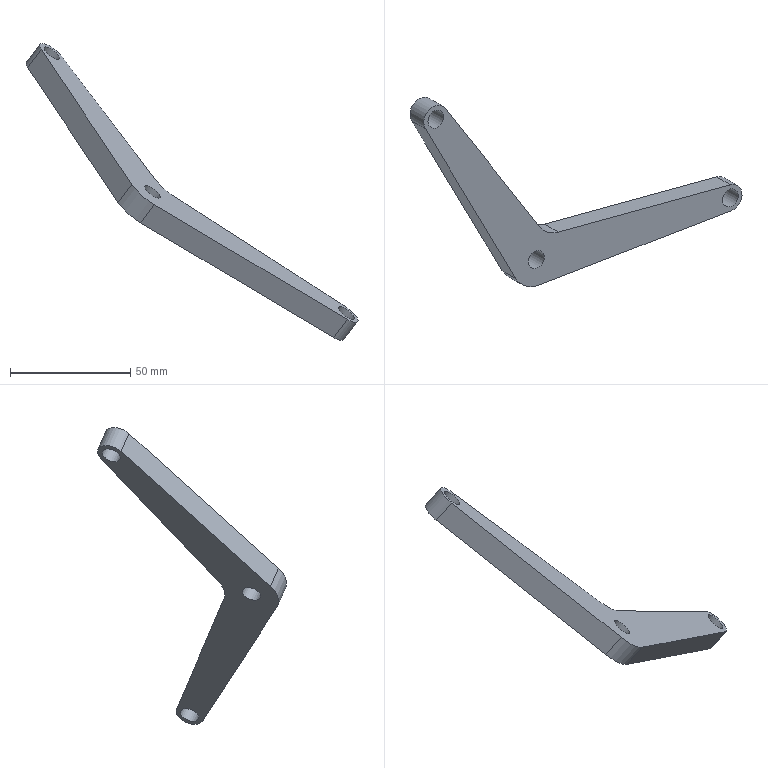Component | NX | QU_BING | 1 solid | 13 faces | box 137.95 x 78.59 x 123.38 mm | volume 32106 mm3 | cylinder 7 | plane 6 | commonest cylinder face diameters 8 x3 24 x2 12.2 x1 11.9 x1
STEP:
#1=CARTESIAN_POINT('',(0.,0.,0.));
#2=DIRECTION('',(0.,0.,1.));
#3=DIRECTION('',(1.,0.,0.));
#4=AXIS2_PLACEMENT_3D('',#1,#2,#3);
#5=CARTESIAN_POINT('',(-160.12,-112.198,24.427));
#6=VERTEX_POINT('',#5);
#7=CARTESIAN_POINT('',(-197.676,-50.115,80.493));
#8=VERTEX_POINT('',#7);
#9=CARTESIAN_POINT('',(-160.12,-112.198,24.427));
#10=DIRECTION('',(-0.4096,0.6771,0.6114));
#11=VECTOR('',#10,1.);
#12=LINE('',#9,#11);
#13=CARTESIAN_POINT('',(-165.855,-108.898,16.93));
#14=DIRECTION('',(0.7094,0.6578,-0.2532));
#15=DIRECTION('',(0.4096,-0.6771,-0.6114));
#16=AXIS2_PLACEMENT_3D('',#13,#14,#15);
#17=PLANE('',#16);
#18=CARTESIAN_POINT('',(0.,-10.));
#19=DIRECTION('',(-1.,-0.));
#20=VECTOR('',#19,1.);
#21=LINE('',#18,#20);
#22=(GEOMETRIC_REPRESENTATION_CONTEXT(2)PARAMETRIC_REPRESENTATION_CONTEXT()REPRESENTATION_CONTEXT('',''));
#23=DEFINITIONAL_REPRESENTATION('',(#21),#22);
#24=PCURVE('',#17,#23);
#25=CARTESIAN_POINT('',(-193.349,-46.103,78.949));
#26=DIRECTION('',(-0.5736,0.3301,-0.7497));
#27=DIRECTION('',(0.7094,0.6578,-0.2532));
#28=AXIS2_PLACEMENT_3D('',#25,#26,#27);
#29=PLANE('',#28);
#30=CARTESIAN_POINT('',(-6.1,91.696));
#31=DIRECTION('',(-0.,-1.));
#32=VECTOR('',#31,1.);
#33=LINE('',#30,#32);
#34=(GEOMETRIC_REPRESENTATION_CONTEXT(2)PARAMETRIC_REPRESENTATION_CONTEXT()REPRESENTATION_CONTEXT('',''));
#35=DEFINITIONAL_REPRESENTATION('',(#33),#34);
#36=PCURVE('',#29,#35);
#37=SURFACE_CURVE('',#12,(#24,#36),.PCURVE_S1.);
#38=EDGE_CURVE('',#6,#8,#37,.T.);
#39=ORIENTED_EDGE('',*,*,#38,.T.);
#40=CARTESIAN_POINT('',(-203.412,-46.814,72.996));
#41=VERTEX_POINT('',#40);
#42=CARTESIAN_POINT('',(-203.412,-46.814,72.996));
#43=DIRECTION('',(0.5736,-0.3301,0.7497));
#44=VECTOR('',#43,1.);
#45=LINE('',#42,#44);
#46=CARTESIAN_POINT('',(-91.696,0.));
#47=DIRECTION('',(0.,-1.));
#48=VECTOR('',#47,1.);
#49=LINE('',#46,#48);
#50=(GEOMETRIC_REPRESENTATION_CONTEXT(2)PARAMETRIC_REPRESENTATION_CONTEXT()REPRESENTATION_CONTEXT('',''));
#51=DEFINITIONAL_REPRESENTATION('',(#49),#50);
#52=PCURVE('',#17,#51);
#53=CARTESIAN_POINT('',(-199.085,-42.802,71.452));
#54=DIRECTION('',(0.5736,-0.3301,0.7497));
#55=DIRECTION('',(-0.7094,-0.6578,0.2532));
#56=AXIS2_PLACEMENT_3D('',#53,#54,#55);
#57=CYLINDRICAL_SURFACE('',#56,6.1);
#58=CARTESIAN_POINT('',(6.283,-0.));
#59=DIRECTION('',(0.,1.));
#60=VECTOR('',#59,1.);
#61=LINE('',#58,#60);
#62=(GEOMETRIC_REPRESENTATION_CONTEXT(2)PARAMETRIC_REPRESENTATION_CONTEXT()REPRESENTATION_CONTEXT('',''));
#63=DEFINITIONAL_REPRESENTATION('',(#61),#62);
#64=PCURVE('',#57,#63);
#65=SURFACE_CURVE('',#45,(#52,#64),.PCURVE_S1.);
#66=EDGE_CURVE('',#41,#8,#65,.T.);
#67=ORIENTED_EDGE('',*,*,#66,.F.);
#68=CARTESIAN_POINT('',(-165.855,-108.898,16.93));
#69=VERTEX_POINT('',#68);
#70=CARTESIAN_POINT('',(-165.855,-108.898,16.93));
#71=DIRECTION('',(-0.4096,0.6771,0.6114));
#72=VECTOR('',#71,1.);
#73=LINE('',#70,#72);
#74=CARTESIAN_POINT('',(0.,0.));
#75=DIRECTION('',(-1.,-0.));
#76=VECTOR('',#75,1.);
#77=LINE('',#74,#76);
#78=(GEOMETRIC_REPRESENTATION_CONTEXT(2)PARAMETRIC_REPRESENTATION_CONTEXT()REPRESENTATION_CONTEXT('',''));
#79=DEFINITIONAL_REPRESENTATION('',(#77),#78);
#80=PCURVE('',#17,#79);
#81=CARTESIAN_POINT('',(-199.085,-42.802,71.452));
#82=DIRECTION('',(-0.5736,0.3301,-0.7497));
#83=DIRECTION('',(0.7094,0.6578,-0.2532));
#84=AXIS2_PLACEMENT_3D('',#81,#82,#83);
#85=PLANE('',#84);
#86=CARTESIAN_POINT('',(-6.1,91.696));
#87=DIRECTION('',(-0.,-1.));
#88=VECTOR('',#87,1.);
#89=LINE('',#86,#88);
#90=(GEOMETRIC_REPRESENTATION_CONTEXT(2)PARAMETRIC_REPRESENTATION_CONTEXT()REPRESENTATION_CONTEXT('',''));
#91=DEFINITIONAL_REPRESENTATION('',(#89),#90);
#92=PCURVE('',#85,#91);
#93=SURFACE_CURVE('',#73,(#80,#92),.PCURVE_S1.);
#94=EDGE_CURVE('',#69,#41,#93,.T.);
#95=ORIENTED_EDGE('',*,*,#94,.F.);
#96=CARTESIAN_POINT('',(-165.855,-108.898,16.93));
#97=DIRECTION('',(0.5736,-0.3301,0.7497));
#98=VECTOR('',#97,1.);
#99=LINE('',#96,#98);
#100=CARTESIAN_POINT('',(0.,0.));
#101=DIRECTION('',(0.,-1.));
#102=VECTOR('',#101,1.);
#103=LINE('',#100,#102);
#104=(GEOMETRIC_REPRESENTATION_CONTEXT(2)PARAMETRIC_REPRESENTATION_CONTEXT()REPRESENTATION_CONTEXT('',''));
#105=DEFINITIONAL_REPRESENTATION('',(#103),#104);
#106=PCURVE('',#17,#105);
#107=CARTESIAN_POINT('',(-157.343,-101.004,13.892));
#108=DIRECTION('',(0.5736,-0.3301,0.7497));
#109=DIRECTION('',(-0.7094,-0.6578,0.2532));
#110=AXIS2_PLACEMENT_3D('',#107,#108,#109);
#111=CYLINDRICAL_SURFACE('',#110,12.);
#112=CARTESIAN_POINT('',(0.,0.));
#113=DIRECTION('',(0.,1.));
#114=VECTOR('',#113,1.);
#115=LINE('',#112,#114);
#116=(GEOMETRIC_REPRESENTATION_CONTEXT(2)PARAMETRIC_REPRESENTATION_CONTEXT()REPRESENTATION_CONTEXT('',''));
#117=DEFINITIONAL_REPRESENTATION('',(#115),#116);
#118=PCURVE('',#111,#117);
#119=SURFACE_CURVE('',#99,(#106,#118),.PCURVE_S1.);
#120=EDGE_CURVE('',#69,#6,#119,.T.);
#121=ORIENTED_EDGE('',*,*,#120,.T.);
#122=EDGE_LOOP('',(#39,#67,#95,#121));
#123=FACE_BOUND('',#122,.T.);
#124=ADVANCED_FACE('',(#123),#17,.F.);
#125=CARTESIAN_POINT('',(-189.306,-41.681,77.803));
#126=VERTEX_POINT('',#125);
#127=CARTESIAN_POINT('',(-193.349,-46.103,78.949));
#128=DIRECTION('',(-0.5736,0.3301,-0.7497));
#129=DIRECTION('',(0.7094,0.6578,-0.2532));
#130=AXIS2_PLACEMENT_3D('',#127,#128,#129);
#131=CIRCLE('',#130,6.1);
#132=CARTESIAN_POINT('',(9.425,10.));
#133=DIRECTION('',(-1.,-0.));
#134=VECTOR('',#133,1.);
#135=LINE('',#132,#134);
#136=(GEOMETRIC_REPRESENTATION_CONTEXT(2)PARAMETRIC_REPRESENTATION_CONTEXT()REPRESENTATION_CONTEXT('',''));
#137=DEFINITIONAL_REPRESENTATION('',(#135),#136);
#138=PCURVE('',#57,#137);
#139=CARTESIAN_POINT('',(0.,0.));
#140=DIRECTION('',(1.,-0.));
#141=AXIS2_PLACEMENT_2D('',#139,#140);
#142=CIRCLE('',#141,6.1);
#143=(GEOMETRIC_REPRESENTATION_CONTEXT(2)PARAMETRIC_REPRESENTATION_CONTEXT()REPRESENTATION_CONTEXT('',''));
#144=DEFINITIONAL_REPRESENTATION('',(#142),#143);
#145=PCURVE('',#29,#144);
#146=SURFACE_CURVE('',#131,(#138,#145),.PCURVE_S1.);
#147=EDGE_CURVE('',#8,#126,#146,.T.);
#148=ORIENTED_EDGE('',*,*,#147,.T.);
#149=CARTESIAN_POINT('',(-195.042,-38.38,70.306));
#150=VERTEX_POINT('',#149);
#151=CARTESIAN_POINT('',(-195.042,-38.38,70.306));
#152=DIRECTION('',(0.5736,-0.3301,0.7497));
#153=VECTOR('',#152,1.);
#154=LINE('',#151,#153);
#155=CARTESIAN_POINT('',(3.246,0.));
#156=DIRECTION('',(0.,1.));
#157=VECTOR('',#156,1.);
#158=LINE('',#155,#157);
#159=(GEOMETRIC_REPRESENTATION_CONTEXT(2)PARAMETRIC_REPRESENTATION_CONTEXT()REPRESENTATION_CONTEXT('',''));
#160=DEFINITIONAL_REPRESENTATION('',(#158),#159);
#161=PCURVE('',#57,#160);
#162=CARTESIAN_POINT('',(-195.042,-38.38,70.306));
#163=DIRECTION('',(-0.6627,-0.7249,0.1879));
#164=DIRECTION('',(-0.4815,0.6046,0.6345));
#165=AXIS2_PLACEMENT_3D('',#162,#163,#164);
#166=PLANE('',#165);
#167=CARTESIAN_POINT('',(0.,0.));
#168=DIRECTION('',(0.,-1.));
#169=VECTOR('',#168,1.);
#170=LINE('',#167,#169);
#171=(GEOMETRIC_REPRESENTATION_CONTEXT(2)PARAMETRIC_REPRESENTATION_CONTEXT()REPRESENTATION_CONTEXT('',''));
#172=DEFINITIONAL_REPRESENTATION('',(#170),#171);
#173=PCURVE('',#166,#172);
#174=SURFACE_CURVE('',#154,(#161,#173),.PCURVE_S1.);
#175=EDGE_CURVE('',#150,#126,#174,.T.);
#176=ORIENTED_EDGE('',*,*,#175,.F.);
#177=CARTESIAN_POINT('',(-199.085,-42.802,71.452));
#178=DIRECTION('',(-0.5736,0.3301,-0.7497));
#179=DIRECTION('',(0.7094,0.6578,-0.2532));
#180=AXIS2_PLACEMENT_3D('',#177,#178,#179);
#181=CIRCLE('',#180,6.1);
#182=CARTESIAN_POINT('',(9.425,0.));
#183=DIRECTION('',(-1.,-0.));
#184=VECTOR('',#183,1.);
#185=LINE('',#182,#184);
#186=(GEOMETRIC_REPRESENTATION_CONTEXT(2)PARAMETRIC_REPRESENTATION_CONTEXT()REPRESENTATION_CONTEXT('',''));
#187=DEFINITIONAL_REPRESENTATION('',(#185),#186);
#188=PCURVE('',#57,#187);
#189=CARTESIAN_POINT('',(0.,0.));
#190=DIRECTION('',(1.,-0.));
#191=AXIS2_PLACEMENT_2D('',#189,#190);
#192=CIRCLE('',#191,6.1);
#193=(GEOMETRIC_REPRESENTATION_CONTEXT(2)PARAMETRIC_REPRESENTATION_CONTEXT()REPRESENTATION_CONTEXT('',''));
#194=DEFINITIONAL_REPRESENTATION('',(#192),#193);
#195=PCURVE('',#85,#194);
#196=SURFACE_CURVE('',#181,(#188,#195),.PCURVE_S1.);
#197=EDGE_CURVE('',#41,#150,#196,.T.);
#198=ORIENTED_EDGE('',*,*,#197,.F.);
#199=ORIENTED_EDGE('',*,*,#66,.T.);
#200=EDGE_LOOP('',(#148,#176,#198,#199));
#201=FACE_BOUND('',#200,.T.);
#202=ADVANCED_FACE('',(#201),#57,.T.);
#203=CARTESIAN_POINT('',(-150.342,-90.607,26.452));
#204=VERTEX_POINT('',#203);
#205=CARTESIAN_POINT('',(-189.306,-41.681,77.803));
#206=DIRECTION('',(0.4815,-0.6046,-0.6345));
#207=VECTOR('',#206,1.);
#208=LINE('',#205,#207);
#209=CARTESIAN_POINT('',(0.,-10.));
#210=DIRECTION('',(-1.,0.));
#211=VECTOR('',#210,1.);
#212=LINE('',#209,#211);
#213=(GEOMETRIC_REPRESENTATION_CONTEXT(2)PARAMETRIC_REPRESENTATION_CONTEXT()REPRESENTATION_CONTEXT('',''));
#214=DEFINITIONAL_REPRESENTATION('',(#212),#213);
#215=PCURVE('',#166,#214);
#216=CARTESIAN_POINT('',(6.067,-0.6376));
#217=DIRECTION('',(0.1045,0.9945));
#218=VECTOR('',#217,1.);
#219=LINE('',#216,#218);
#220=(GEOMETRIC_REPRESENTATION_CONTEXT(2)PARAMETRIC_REPRESENTATION_CONTEXT()REPRESENTATION_CONTEXT('',''));
#221=DEFINITIONAL_REPRESENTATION('',(#219),#220);
#222=PCURVE('',#29,#221);
#223=SURFACE_CURVE('',#208,(#215,#222),.PCURVE_S1.);
#224=EDGE_CURVE('',#126,#204,#223,.T.);
#225=ORIENTED_EDGE('',*,*,#224,.T.);
#226=CARTESIAN_POINT('',(-156.078,-87.306,18.955));
#227=VERTEX_POINT('',#226);
#228=CARTESIAN_POINT('',(-156.078,-87.306,18.955));
#229=DIRECTION('',(0.5736,-0.3301,0.7497));
#230=VECTOR('',#229,1.);
#231=LINE('',#228,#230);
#232=CARTESIAN_POINT('',(-80.925,0.));
#233=DIRECTION('',(0.,-1.));
#234=VECTOR('',#233,1.);
#235=LINE('',#232,#234);
#236=(GEOMETRIC_REPRESENTATION_CONTEXT(2)PARAMETRIC_REPRESENTATION_CONTEXT()REPRESENTATION_CONTEXT('',''));
#237=DEFINITIONAL_REPRESENTATION('',(#235),#236);
#238=PCURVE('',#166,#237);
#239=CARTESIAN_POINT('',(-148.125,-78.607,16.701));
#240=DIRECTION('',(0.5736,-0.3301,0.7497));
#241=DIRECTION('',(-0.7094,-0.6578,0.2532));
#242=AXIS2_PLACEMENT_3D('',#239,#240,#241);
#243=CYLINDRICAL_SURFACE('',#242,12.);
#244=CARTESIAN_POINT('',(0.1047,-0.));
#245=DIRECTION('',(0.,1.));
#246=VECTOR('',#245,1.);
#247=LINE('',#244,#246);
#248=(GEOMETRIC_REPRESENTATION_CONTEXT(2)PARAMETRIC_REPRESENTATION_CONTEXT()REPRESENTATION_CONTEXT('',''));
#249=DEFINITIONAL_REPRESENTATION('',(#247),#248);
#250=PCURVE('',#243,#249);
#251=SURFACE_CURVE('',#231,(#238,#250),.PCURVE_S1.);
#252=EDGE_CURVE('',#227,#204,#251,.T.);
#253=ORIENTED_EDGE('',*,*,#252,.F.);
#254=CARTESIAN_POINT('',(-195.042,-38.38,70.306));
#255=DIRECTION('',(0.4815,-0.6046,-0.6345));
#256=VECTOR('',#255,1.);
#257=LINE('',#254,#256);
#258=CARTESIAN_POINT('',(0.,0.));
#259=DIRECTION('',(-1.,0.));
#260=VECTOR('',#259,1.);
#261=LINE('',#258,#260);
#262=(GEOMETRIC_REPRESENTATION_CONTEXT(2)PARAMETRIC_REPRESENTATION_CONTEXT()REPRESENTATION_CONTEXT('',''));
#263=DEFINITIONAL_REPRESENTATION('',(#261),#262);
#264=PCURVE('',#166,#263);
#265=CARTESIAN_POINT('',(6.067,-0.6376));
#266=DIRECTION('',(0.1045,0.9945));
#267=VECTOR('',#266,1.);
#268=LINE('',#265,#267);
#269=(GEOMETRIC_REPRESENTATION_CONTEXT(2)PARAMETRIC_REPRESENTATION_CONTEXT()REPRESENTATION_CONTEXT('',''));
#270=DEFINITIONAL_REPRESENTATION('',(#268),#269);
#271=PCURVE('',#85,#270);
#272=SURFACE_CURVE('',#257,(#264,#271),.PCURVE_S1.);
#273=EDGE_CURVE('',#150,#227,#272,.T.);
#274=ORIENTED_EDGE('',*,*,#273,.F.);
#275=ORIENTED_EDGE('',*,*,#175,.T.);
#276=EDGE_LOOP('',(#225,#253,#274,#275));
#277=FACE_BOUND('',#276,.T.);
#278=ADVANCED_FACE('',(#277),#166,.F.);
#279=ORIENTED_EDGE('',*,*,#252,.F.);
#280=CARTESIAN_POINT('',(-148.177,-89.604,11.899));
#281=VERTEX_POINT('',#280);
#282=CARTESIAN_POINT('',(-148.125,-78.607,16.701));
#283=DIRECTION('',(0.5736,-0.3301,0.7497));
#284=DIRECTION('',(0.7094,0.6578,-0.2532));
#285=AXIS2_PLACEMENT_3D('',#282,#283,#284);
#286=CIRCLE('',#285,12.);
#287=CARTESIAN_POINT('',(-3.142,-0.));
#288=DIRECTION('',(1.,0.));
#289=VECTOR('',#288,1.);
#290=LINE('',#287,#289);
#291=(GEOMETRIC_REPRESENTATION_CONTEXT(2)PARAMETRIC_REPRESENTATION_CONTEXT()REPRESENTATION_CONTEXT('',''));
#292=DEFINITIONAL_REPRESENTATION('',(#290),#291);
#293=PCURVE('',#243,#292);
#294=CARTESIAN_POINT('',(38.46,78.59));
#295=CARTESIAN_POINT('',(38.46,57.805));
#296=CARTESIAN_POINT('',(20.46,68.198));
#297=CARTESIAN_POINT('',(2.46,78.59));
#298=CARTESIAN_POINT('',(20.46,88.982));
#299=CARTESIAN_POINT('',(38.46,99.375));
#300=CARTESIAN_POINT('',(38.46,78.59));
#301=(BOUNDED_CURVE()B_SPLINE_CURVE(2,(#294,#295,#296,#297,#298,#299,#300),.UNSPECIFIED.,.T.,.F.)B_SPLINE_CURVE_WITH_KNOTS((1,2,2,2,2,1),(-2.094,0.,2.094,4.189,6.283,8.378),.UNSPECIFIED.)CURVE()GEOMETRIC_REPRESENTATION_ITEM()RATIONAL_B_SPLINE_CURVE((1.,0.5,1.,0.5,1.,0.5,1.))REPRESENTATION_ITEM(''));
#302=(GEOMETRIC_REPRESENTATION_CONTEXT(2)PARAMETRIC_REPRESENTATION_CONTEXT()REPRESENTATION_CONTEXT('',''));
#303=DEFINITIONAL_REPRESENTATION('',(#301),#302);
#304=PCURVE('',#85,#303);
#305=SURFACE_CURVE('',#286,(#293,#304),.PCURVE_S1.);
#306=EDGE_CURVE('',#227,#281,#305,.T.);
#307=ORIENTED_EDGE('',*,*,#306,.T.);
#308=CARTESIAN_POINT('',(-142.441,-92.905,19.396));
#309=VERTEX_POINT('',#308);
#310=CARTESIAN_POINT('',(-148.177,-89.604,11.899));
#311=DIRECTION('',(0.5736,-0.3301,0.7497));
#312=VECTOR('',#311,1.);
#313=LINE('',#310,#312);
#314=CARTESIAN_POINT('',(1.042,-0.));
#315=DIRECTION('',(0.,1.));
#316=VECTOR('',#315,1.);
#317=LINE('',#314,#316);
#318=(GEOMETRIC_REPRESENTATION_CONTEXT(2)PARAMETRIC_REPRESENTATION_CONTEXT()REPRESENTATION_CONTEXT('',''));
#319=DEFINITIONAL_REPRESENTATION('',(#317),#318);
#320=PCURVE('',#243,#319);
#321=CARTESIAN_POINT('',(-148.177,-89.604,11.899));
#322=DIRECTION('',(-0.004289,-0.9164,-0.4002));
#323=DIRECTION('',(-0.8191,-0.2263,0.5271));
#324=AXIS2_PLACEMENT_3D('',#321,#322,#323);
#325=PLANE('',#324);
#326=CARTESIAN_POINT('',(0.,0.));
#327=DIRECTION('',(0.,-1.));
#328=VECTOR('',#327,1.);
#329=LINE('',#326,#328);
#330=(GEOMETRIC_REPRESENTATION_CONTEXT(2)PARAMETRIC_REPRESENTATION_CONTEXT()REPRESENTATION_CONTEXT('',''));
#331=DEFINITIONAL_REPRESENTATION('',(#329),#330);
#332=PCURVE('',#325,#331);
#333=SURFACE_CURVE('',#313,(#320,#332),.PCURVE_S1.);
#334=EDGE_CURVE('',#281,#309,#333,.T.);
#335=ORIENTED_EDGE('',*,*,#334,.T.);
#336=CARTESIAN_POINT('',(-142.389,-81.908,24.198));
#337=DIRECTION('',(0.5736,-0.3301,0.7497));
#338=DIRECTION('',(0.7094,0.6578,-0.2532));
#339=AXIS2_PLACEMENT_3D('',#336,#337,#338);
#340=CIRCLE('',#339,12.);
#341=CARTESIAN_POINT('',(-3.142,10.));
#342=DIRECTION('',(1.,0.));
#343=VECTOR('',#342,1.);
#344=LINE('',#341,#343);
#345=(GEOMETRIC_REPRESENTATION_CONTEXT(2)PARAMETRIC_REPRESENTATION_CONTEXT()REPRESENTATION_CONTEXT('',''));
#346=DEFINITIONAL_REPRESENTATION('',(#344),#345);
#347=PCURVE('',#243,#346);
#348=CARTESIAN_POINT('',(38.46,78.59));
#349=CARTESIAN_POINT('',(38.46,57.805));
#350=CARTESIAN_POINT('',(20.46,68.198));
#351=CARTESIAN_POINT('',(2.46,78.59));
#352=CARTESIAN_POINT('',(20.46,88.982));
#353=CARTESIAN_POINT('',(38.46,99.375));
#354=CARTESIAN_POINT('',(38.46,78.59));
#355=(BOUNDED_CURVE()B_SPLINE_CURVE(2,(#348,#349,#350,#351,#352,#353,#354),.UNSPECIFIED.,.T.,.F.)B_SPLINE_CURVE_WITH_KNOTS((1,2,2,2,2,1),(-2.094,0.,2.094,4.189,6.283,8.378),.UNSPECIFIED.)CURVE()GEOMETRIC_REPRESENTATION_ITEM()RATIONAL_B_SPLINE_CURVE((1.,0.5,1.,0.5,1.,0.5,1.))REPRESENTATION_ITEM(''));
#356=(GEOMETRIC_REPRESENTATION_CONTEXT(2)PARAMETRIC_REPRESENTATION_CONTEXT()REPRESENTATION_CONTEXT('',''));
#357=DEFINITIONAL_REPRESENTATION('',(#355),#356);
#358=PCURVE('',#29,#357);
#359=SURFACE_CURVE('',#340,(#347,#358),.PCURVE_S1.);
#360=EDGE_CURVE('',#204,#309,#359,.T.);
#361=ORIENTED_EDGE('',*,*,#360,.F.);
#362=EDGE_LOOP('',(#279,#307,#335,#361));
#363=FACE_BOUND('',#362,.F.);
#364=ADVANCED_FACE('',(#363),#243,.F.);
#365=CARTESIAN_POINT('',(-70.984,-73.162,-26.581));
#366=VERTEX_POINT('',#365);
#367=CARTESIAN_POINT('',(-142.441,-92.905,19.396));
#368=DIRECTION('',(0.8191,0.2263,-0.5271));
#369=VECTOR('',#368,1.);
#370=LINE('',#367,#369);
#371=CARTESIAN_POINT('',(0.,-10.));
#372=DIRECTION('',(-1.,-0.));
#373=VECTOR('',#372,1.);
#374=LINE('',#371,#373);
#375=(GEOMETRIC_REPRESENTATION_CONTEXT(2)PARAMETRIC_REPRESENTATION_CONTEXT()REPRESENTATION_CONTEXT('',''));
#376=DEFINITIONAL_REPRESENTATION('',(#374),#375);
#377=PCURVE('',#325,#376);
#378=CARTESIAN_POINT('',(20.406,88.951));
#379=DIRECTION('',(0.8634,0.5045));
#380=VECTOR('',#379,1.);
#381=LINE('',#378,#380);
#382=(GEOMETRIC_REPRESENTATION_CONTEXT(2)PARAMETRIC_REPRESENTATION_CONTEXT()REPRESENTATION_CONTEXT('',''));
#383=DEFINITIONAL_REPRESENTATION('',(#381),#382);
#384=PCURVE('',#29,#383);
#385=SURFACE_CURVE('',#370,(#377,#384),.PCURVE_S1.);
#386=EDGE_CURVE('',#309,#366,#385,.T.);
#387=ORIENTED_EDGE('',*,*,#386,.T.);
#388=CARTESIAN_POINT('',(-76.72,-69.861,-34.078));
#389=VERTEX_POINT('',#388);
#390=CARTESIAN_POINT('',(-76.72,-69.861,-34.078));
#391=DIRECTION('',(0.5736,-0.3301,0.7497));
#392=VECTOR('',#391,1.);
#393=LINE('',#390,#392);
#394=CARTESIAN_POINT('',(-87.234,0.));
#395=DIRECTION('',(0.,-1.));
#396=VECTOR('',#395,1.);
#397=LINE('',#394,#396);
#398=(GEOMETRIC_REPRESENTATION_CONTEXT(2)PARAMETRIC_REPRESENTATION_CONTEXT()REPRESENTATION_CONTEXT('',''));
#399=DEFINITIONAL_REPRESENTATION('',(#397),#398);
#400=PCURVE('',#325,#399);
#401=CARTESIAN_POINT('',(-76.745,-75.314,-36.459));
#402=DIRECTION('',(0.5736,-0.3301,0.7497));
#403=DIRECTION('',(-0.7094,-0.6578,0.2532));
#404=AXIS2_PLACEMENT_3D('',#401,#402,#403);
#405=CYLINDRICAL_SURFACE('',#404,5.95);
#406=CARTESIAN_POINT('',(4.184,0.));
#407=DIRECTION('',(-0.,1.));
#408=VECTOR('',#407,1.);
#409=LINE('',#406,#408);
#410=(GEOMETRIC_REPRESENTATION_CONTEXT(2)PARAMETRIC_REPRESENTATION_CONTEXT()REPRESENTATION_CONTEXT('',''));
#411=DEFINITIONAL_REPRESENTATION('',(#409),#410);
#412=PCURVE('',#405,#411);
#413=SURFACE_CURVE('',#393,(#400,#412),.PCURVE_S1.);
#414=EDGE_CURVE('',#389,#366,#413,.T.);
#415=ORIENTED_EDGE('',*,*,#414,.F.);
#416=CARTESIAN_POINT('',(-148.177,-89.604,11.899));
#417=DIRECTION('',(0.8191,0.2263,-0.5271));
#418=VECTOR('',#417,1.);
#419=LINE('',#416,#418);
#420=CARTESIAN_POINT('',(0.,0.));
#421=DIRECTION('',(-1.,-0.));
#422=VECTOR('',#421,1.);
#423=LINE('',#420,#422);
#424=(GEOMETRIC_REPRESENTATION_CONTEXT(2)PARAMETRIC_REPRESENTATION_CONTEXT()REPRESENTATION_CONTEXT('',''));
#425=DEFINITIONAL_REPRESENTATION('',(#423),#424);
#426=PCURVE('',#325,#425);
#427=CARTESIAN_POINT('',(20.406,88.951));
#428=DIRECTION('',(0.8634,0.5045));
#429=VECTOR('',#428,1.);
#430=LINE('',#427,#429);
#431=(GEOMETRIC_REPRESENTATION_CONTEXT(2)PARAMETRIC_REPRESENTATION_CONTEXT()REPRESENTATION_CONTEXT('',''));
#432=DEFINITIONAL_REPRESENTATION('',(#430),#431);
#433=PCURVE('',#85,#432);
#434=SURFACE_CURVE('',#419,(#426,#433),.PCURVE_S1.);
#435=EDGE_CURVE('',#281,#389,#434,.T.);
#436=ORIENTED_EDGE('',*,*,#435,.F.);
#437=ORIENTED_EDGE('',*,*,#334,.T.);
#438=EDGE_LOOP('',(#387,#415,#436,#437));
#439=FACE_BOUND('',#438,.T.);
#440=ADVANCED_FACE('',(#439),#325,.F.);
#441=CARTESIAN_POINT('',(-70.551,-83.907,-31.643));
#442=VERTEX_POINT('',#441);
#443=CARTESIAN_POINT('',(-71.01,-78.615,-28.962));
#444=DIRECTION('',(-0.5736,0.3301,-0.7497));
#445=DIRECTION('',(0.7094,0.6578,-0.2532));
#446=AXIS2_PLACEMENT_3D('',#443,#444,#445);
#447=CIRCLE('',#446,5.95);
#448=CARTESIAN_POINT('',(9.425,10.));
#449=DIRECTION('',(-1.,0.));
#450=VECTOR('',#449,1.);
#451=LINE('',#448,#450);
#452=(GEOMETRIC_REPRESENTATION_CONTEXT(2)PARAMETRIC_REPRESENTATION_CONTEXT()REPRESENTATION_CONTEXT('',''));
#453=DEFINITIONAL_REPRESENTATION('',(#451),#452);
#454=PCURVE('',#405,#453);
#455=CARTESIAN_POINT('',(92.721,138.1));
#456=DIRECTION('',(1.,-0.));
#457=AXIS2_PLACEMENT_2D('',#455,#456);
#458=CIRCLE('',#457,5.95);
#459=(GEOMETRIC_REPRESENTATION_CONTEXT(2)PARAMETRIC_REPRESENTATION_CONTEXT()REPRESENTATION_CONTEXT('',''));
#460=DEFINITIONAL_REPRESENTATION('',(#458),#459);
#461=PCURVE('',#29,#460);
#462=SURFACE_CURVE('',#447,(#454,#461),.PCURVE_S1.);
#463=EDGE_CURVE('',#366,#442,#462,.T.);
#464=ORIENTED_EDGE('',*,*,#463,.T.);
#465=CARTESIAN_POINT('',(-76.287,-80.606,-39.14));
#466=VERTEX_POINT('',#465);
#467=CARTESIAN_POINT('',(-76.287,-80.606,-39.14));
#468=DIRECTION('',(0.5736,-0.3301,0.7497));
#469=VECTOR('',#468,1.);
#470=LINE('',#467,#469);
#471=CARTESIAN_POINT('',(1.141,0.));
#472=DIRECTION('',(0.,1.));
#473=VECTOR('',#472,1.);
#474=LINE('',#471,#473);
#475=(GEOMETRIC_REPRESENTATION_CONTEXT(2)PARAMETRIC_REPRESENTATION_CONTEXT()REPRESENTATION_CONTEXT('',''));
#476=DEFINITIONAL_REPRESENTATION('',(#474),#475);
#477=PCURVE('',#405,#476);
#478=CARTESIAN_POINT('',(-76.287,-80.606,-39.14));
#479=DIRECTION('',(-0.07709,0.8894,0.4506));
#480=DIRECTION('',(0.8155,0.3162,-0.4847));
#481=AXIS2_PLACEMENT_3D('',#478,#479,#480);
#482=PLANE('',#481);
#483=CARTESIAN_POINT('',(-0.,0.));
#484=DIRECTION('',(-0.,-1.));
#485=VECTOR('',#484,1.);
#486=LINE('',#483,#485);
#487=(GEOMETRIC_REPRESENTATION_CONTEXT(2)PARAMETRIC_REPRESENTATION_CONTEXT()REPRESENTATION_CONTEXT('',''));
#488=DEFINITIONAL_REPRESENTATION('',(#486),#487);
#489=PCURVE('',#482,#488);
#490=SURFACE_CURVE('',#470,(#477,#489),.PCURVE_S1.);
#491=EDGE_CURVE('',#466,#442,#490,.T.);
#492=ORIENTED_EDGE('',*,*,#491,.F.);
#493=CARTESIAN_POINT('',(-76.745,-75.314,-36.459));
#494=DIRECTION('',(-0.5736,0.3301,-0.7497));
#495=DIRECTION('',(0.7094,0.6578,-0.2532));
#496=AXIS2_PLACEMENT_3D('',#493,#494,#495);
#497=CIRCLE('',#496,5.95);
#498=CARTESIAN_POINT('',(9.425,0.));
#499=DIRECTION('',(-1.,0.));
#500=VECTOR('',#499,1.);
#501=LINE('',#498,#500);
#502=(GEOMETRIC_REPRESENTATION_CONTEXT(2)PARAMETRIC_REPRESENTATION_CONTEXT()REPRESENTATION_CONTEXT('',''));
#503=DEFINITIONAL_REPRESENTATION('',(#501),#502);
#504=PCURVE('',#405,#503);
#505=CARTESIAN_POINT('',(92.721,138.1));
#506=DIRECTION('',(1.,-0.));
#507=AXIS2_PLACEMENT_2D('',#505,#506);
#508=CIRCLE('',#507,5.95);
#509=(GEOMETRIC_REPRESENTATION_CONTEXT(2)PARAMETRIC_REPRESENTATION_CONTEXT()REPRESENTATION_CONTEXT('',''));
#510=DEFINITIONAL_REPRESENTATION('',(#508),#509);
#511=PCURVE('',#85,#510);
#512=SURFACE_CURVE('',#497,(#504,#511),.PCURVE_S1.);
#513=EDGE_CURVE('',#389,#466,#512,.T.);
#514=ORIENTED_EDGE('',*,*,#513,.F.);
#515=ORIENTED_EDGE('',*,*,#414,.T.);
#516=EDGE_LOOP('',(#464,#492,#514,#515));
#517=FACE_BOUND('',#516,.T.);
#518=ADVANCED_FACE('',(#517),#405,.T.);
#519=CARTESIAN_POINT('',(-150.682,-114.978,15.983));
#520=VERTEX_POINT('',#519);
#521=CARTESIAN_POINT('',(-70.551,-83.907,-31.643));
#522=DIRECTION('',(-0.8155,-0.3162,0.4847));
#523=VECTOR('',#522,1.);
#524=LINE('',#521,#523);
#525=CARTESIAN_POINT('',(-0.,-10.));
#526=DIRECTION('',(-1.,0.));
#527=VECTOR('',#526,1.);
#528=LINE('',#525,#527);
#529=(GEOMETRIC_REPRESENTATION_CONTEXT(2)PARAMETRIC_REPRESENTATION_CONTEXT()REPRESENTATION_CONTEXT('',''));
#530=DEFINITIONAL_REPRESENTATION('',(#528),#529);
#531=PCURVE('',#482,#530);
#532=CARTESIAN_POINT('',(90.244,143.51));
#533=DIRECTION('',(-0.9092,-0.4163));
#534=VECTOR('',#533,1.);
#535=LINE('',#532,#534);
#536=(GEOMETRIC_REPRESENTATION_CONTEXT(2)PARAMETRIC_REPRESENTATION_CONTEXT()REPRESENTATION_CONTEXT('',''));
#537=DEFINITIONAL_REPRESENTATION('',(#535),#536);
#538=PCURVE('',#29,#537);
#539=SURFACE_CURVE('',#524,(#531,#538),.PCURVE_S1.);
#540=EDGE_CURVE('',#442,#520,#539,.T.);
#541=ORIENTED_EDGE('',*,*,#540,.T.);
#542=CARTESIAN_POINT('',(-156.417,-111.677,8.486));
#543=VERTEX_POINT('',#542);
#544=CARTESIAN_POINT('',(-156.417,-111.677,8.486));
#545=DIRECTION('',(0.5736,-0.3301,0.7497));
#546=VECTOR('',#545,1.);
#547=LINE('',#544,#546);
#548=CARTESIAN_POINT('',(-98.258,-0.));
#549=DIRECTION('',(-0.,-1.));
#550=VECTOR('',#549,1.);
#551=LINE('',#548,#550);
#552=(GEOMETRIC_REPRESENTATION_CONTEXT(2)PARAMETRIC_REPRESENTATION_CONTEXT()REPRESENTATION_CONTEXT('',''));
#553=DEFINITIONAL_REPRESENTATION('',(#551),#552);
#554=PCURVE('',#482,#553);
#555=CARTESIAN_POINT('',(1.141,0.));
#556=DIRECTION('',(-0.,1.));
#557=VECTOR('',#556,1.);
#558=LINE('',#555,#557);
#559=(GEOMETRIC_REPRESENTATION_CONTEXT(2)PARAMETRIC_REPRESENTATION_CONTEXT()REPRESENTATION_CONTEXT('',''));
#560=DEFINITIONAL_REPRESENTATION('',(#558),#559);
#561=PCURVE('',#111,#560);
#562=SURFACE_CURVE('',#547,(#554,#561),.PCURVE_S1.);
#563=EDGE_CURVE('',#543,#520,#562,.T.);
#564=ORIENTED_EDGE('',*,*,#563,.F.);
#565=CARTESIAN_POINT('',(-76.287,-80.606,-39.14));
#566=DIRECTION('',(-0.8155,-0.3162,0.4847));
#567=VECTOR('',#566,1.);
#568=LINE('',#565,#567);
#569=CARTESIAN_POINT('',(0.,0.));
#570=DIRECTION('',(-1.,0.));
#571=VECTOR('',#570,1.);
#572=LINE('',#569,#571);
#573=(GEOMETRIC_REPRESENTATION_CONTEXT(2)PARAMETRIC_REPRESENTATION_CONTEXT()REPRESENTATION_CONTEXT('',''));
#574=DEFINITIONAL_REPRESENTATION('',(#572),#573);
#575=PCURVE('',#482,#574);
#576=CARTESIAN_POINT('',(90.244,143.51));
#577=DIRECTION('',(-0.9092,-0.4163));
#578=VECTOR('',#577,1.);
#579=LINE('',#576,#578);
#580=(GEOMETRIC_REPRESENTATION_CONTEXT(2)PARAMETRIC_REPRESENTATION_CONTEXT()REPRESENTATION_CONTEXT('',''));
#581=DEFINITIONAL_REPRESENTATION('',(#579),#580);
#582=PCURVE('',#85,#581);
#583=SURFACE_CURVE('',#568,(#575,#582),.PCURVE_S1.);
#584=EDGE_CURVE('',#466,#543,#583,.T.);
#585=ORIENTED_EDGE('',*,*,#584,.F.);
#586=ORIENTED_EDGE('',*,*,#491,.T.);
#587=EDGE_LOOP('',(#541,#564,#585,#586));
#588=FACE_BOUND('',#587,.T.);
#589=ADVANCED_FACE('',(#588),#482,.F.);
#590=CARTESIAN_POINT('',(-154.505,-98.373,12.88));
#591=VERTEX_POINT('',#590);
#592=CARTESIAN_POINT('',(-157.343,-101.004,13.892));
#593=DIRECTION('',(-0.5736,0.3301,-0.7497));
#594=DIRECTION('',(0.7094,0.6578,-0.2532));
#595=AXIS2_PLACEMENT_3D('',#592,#593,#594);
#596=CIRCLE('',#595,4.);
#597=CARTESIAN_POINT('',(-157.343,-101.004,13.892));
#598=DIRECTION('',(0.5736,-0.3301,0.7497));
#599=DIRECTION('',(-0.7094,-0.6578,0.2532));
#600=AXIS2_PLACEMENT_3D('',#597,#598,#599);
#601=CYLINDRICAL_SURFACE('',#600,4.);
#602=CARTESIAN_POINT('',(9.425,0.));
#603=DIRECTION('',(-1.,0.));
#604=VECTOR('',#603,1.);
#605=LINE('',#602,#604);
#606=(GEOMETRIC_REPRESENTATION_CONTEXT(2)PARAMETRIC_REPRESENTATION_CONTEXT()REPRESENTATION_CONTEXT('',''));
#607=DEFINITIONAL_REPRESENTATION('',(#605),#606);
#608=PCURVE('',#601,#607);
#609=CARTESIAN_POINT('',(5.9,91.696));
#610=DIRECTION('',(1.,0.));
#611=AXIS2_PLACEMENT_2D('',#609,#610);
#612=CIRCLE('',#611,4.);
#613=(GEOMETRIC_REPRESENTATION_CONTEXT(2)PARAMETRIC_REPRESENTATION_CONTEXT()REPRESENTATION_CONTEXT('',''));
#614=DEFINITIONAL_REPRESENTATION('',(#612),#613);
#615=PCURVE('',#85,#614);
#616=SURFACE_CURVE('',#596,(#608,#615),.PCURVE_S1.);
#617=EDGE_CURVE('',#591,#591,#616,.T.);
#618=ORIENTED_EDGE('',*,*,#617,.F.);
#619=CARTESIAN_POINT('',(-148.769,-101.674,20.377));
#620=VERTEX_POINT('',#619);
#621=CARTESIAN_POINT('',(-154.505,-98.373,12.88));
#622=CARTESIAN_POINT('',(-148.769,-101.674,20.377));
#623=B_SPLINE_CURVE_WITH_KNOTS('',1,(#621,#622),.UNSPECIFIED.,.F.,.F.,(2,2),(0.,10.),.PIECEWISE_BEZIER_KNOTS.);
#624=CARTESIAN_POINT('',(9.425,0.));
#625=DIRECTION('',(0.,1.));
#626=VECTOR('',#625,1.);
#627=LINE('',#624,#626);
#628=(GEOMETRIC_REPRESENTATION_CONTEXT(2)PARAMETRIC_REPRESENTATION_CONTEXT()REPRESENTATION_CONTEXT('',''));
#629=DEFINITIONAL_REPRESENTATION('',(#627),#628);
#630=PCURVE('',#601,#629);
#631=CARTESIAN_POINT('',(3.142,0.));
#632=DIRECTION('',(0.,1.));
#633=VECTOR('',#632,1.);
#634=LINE('',#631,#633);
#635=(GEOMETRIC_REPRESENTATION_CONTEXT(2)PARAMETRIC_REPRESENTATION_CONTEXT()REPRESENTATION_CONTEXT('',''));
#636=DEFINITIONAL_REPRESENTATION('',(#634),#635);
#637=PCURVE('',#601,#636);
#638=SEAM_CURVE('',#623,(#630,#637),.PCURVE_S1.);
#639=EDGE_CURVE('',#591,#620,#638,.T.);
#640=ORIENTED_EDGE('',*,*,#639,.T.);
#641=CARTESIAN_POINT('',(-151.607,-104.305,21.389));
#642=DIRECTION('',(-0.5736,0.3301,-0.7497));
#643=DIRECTION('',(0.7094,0.6578,-0.2532));
#644=AXIS2_PLACEMENT_3D('',#641,#642,#643);
#645=CIRCLE('',#644,4.);
#646=CARTESIAN_POINT('',(9.425,10.));
#647=DIRECTION('',(-1.,0.));
#648=VECTOR('',#647,1.);
#649=LINE('',#646,#648);
#650=(GEOMETRIC_REPRESENTATION_CONTEXT(2)PARAMETRIC_REPRESENTATION_CONTEXT()REPRESENTATION_CONTEXT('',''));
#651=DEFINITIONAL_REPRESENTATION('',(#649),#650);
#652=PCURVE('',#601,#651);
#653=CARTESIAN_POINT('',(5.9,91.696));
#654=DIRECTION('',(1.,0.));
#655=AXIS2_PLACEMENT_2D('',#653,#654);
#656=CIRCLE('',#655,4.);
#657=(GEOMETRIC_REPRESENTATION_CONTEXT(2)PARAMETRIC_REPRESENTATION_CONTEXT()REPRESENTATION_CONTEXT('',''));
#658=DEFINITIONAL_REPRESENTATION('',(#656),#657);
#659=PCURVE('',#29,#658);
#660=SURFACE_CURVE('',#645,(#652,#659),.PCURVE_S1.);
#661=EDGE_CURVE('',#620,#620,#660,.T.);
#662=ORIENTED_EDGE('',*,*,#661,.T.);
#663=ORIENTED_EDGE('',*,*,#639,.F.);
#664=EDGE_LOOP('',(#618,#640,#662,#663));
#665=FACE_BOUND('',#664,.F.);
#666=ADVANCED_FACE('',(#665),#601,.F.);
#667=CARTESIAN_POINT('',(-196.247,-40.171,70.439));
#668=VERTEX_POINT('',#667);
#669=CARTESIAN_POINT('',(-199.085,-42.802,71.452));
#670=DIRECTION('',(-0.5736,0.3301,-0.7497));
#671=DIRECTION('',(0.7094,0.6578,-0.2532));
#672=AXIS2_PLACEMENT_3D('',#669,#670,#671);
#673=CIRCLE('',#672,4.);
#674=CARTESIAN_POINT('',(-199.085,-42.802,71.452));
#675=DIRECTION('',(0.5736,-0.3301,0.7497));
#676=DIRECTION('',(-0.7094,-0.6578,0.2532));
#677=AXIS2_PLACEMENT_3D('',#674,#675,#676);
#678=CYLINDRICAL_SURFACE('',#677,4.);
#679=CARTESIAN_POINT('',(9.425,0.));
#680=DIRECTION('',(-1.,0.));
#681=VECTOR('',#680,1.);
#682=LINE('',#679,#681);
#683=(GEOMETRIC_REPRESENTATION_CONTEXT(2)PARAMETRIC_REPRESENTATION_CONTEXT()REPRESENTATION_CONTEXT('',''));
#684=DEFINITIONAL_REPRESENTATION('',(#682),#683);
#685=PCURVE('',#678,#684);
#686=CARTESIAN_POINT('',(0.,0.));
#687=DIRECTION('',(1.,0.));
#688=AXIS2_PLACEMENT_2D('',#686,#687);
#689=CIRCLE('',#688,4.);
#690=(GEOMETRIC_REPRESENTATION_CONTEXT(2)PARAMETRIC_REPRESENTATION_CONTEXT()REPRESENTATION_CONTEXT('',''));
#691=DEFINITIONAL_REPRESENTATION('',(#689),#690);
#692=PCURVE('',#85,#691);
#693=SURFACE_CURVE('',#673,(#685,#692),.PCURVE_S1.);
#694=EDGE_CURVE('',#668,#668,#693,.T.);
#695=ORIENTED_EDGE('',*,*,#694,.F.);
#696=CARTESIAN_POINT('',(-190.511,-43.472,77.936));
#697=VERTEX_POINT('',#696);
#698=CARTESIAN_POINT('',(-196.247,-40.171,70.439));
#699=CARTESIAN_POINT('',(-190.511,-43.472,77.936));
#700=B_SPLINE_CURVE_WITH_KNOTS('',1,(#698,#699),.UNSPECIFIED.,.F.,.F.,(2,2),(0.,10.),.PIECEWISE_BEZIER_KNOTS.);
#701=CARTESIAN_POINT('',(9.425,0.));
#702=DIRECTION('',(0.,1.));
#703=VECTOR('',#702,1.);
#704=LINE('',#701,#703);
#705=(GEOMETRIC_REPRESENTATION_CONTEXT(2)PARAMETRIC_REPRESENTATION_CONTEXT()REPRESENTATION_CONTEXT('',''));
#706=DEFINITIONAL_REPRESENTATION('',(#704),#705);
#707=PCURVE('',#678,#706);
#708=CARTESIAN_POINT('',(3.142,0.));
#709=DIRECTION('',(0.,1.));
#710=VECTOR('',#709,1.);
#711=LINE('',#708,#710);
#712=(GEOMETRIC_REPRESENTATION_CONTEXT(2)PARAMETRIC_REPRESENTATION_CONTEXT()REPRESENTATION_CONTEXT('',''));
#713=DEFINITIONAL_REPRESENTATION('',(#711),#712);
#714=PCURVE('',#678,#713);
#715=SEAM_CURVE('',#700,(#707,#714),.PCURVE_S1.);
#716=EDGE_CURVE('',#668,#697,#715,.T.);
#717=ORIENTED_EDGE('',*,*,#716,.T.);
#718=CARTESIAN_POINT('',(-193.349,-46.103,78.949));
#719=DIRECTION('',(-0.5736,0.3301,-0.7497));
#720=DIRECTION('',(0.7094,0.6578,-0.2532));
#721=AXIS2_PLACEMENT_3D('',#718,#719,#720);
#722=CIRCLE('',#721,4.);
#723=CARTESIAN_POINT('',(9.425,10.));
#724=DIRECTION('',(-1.,0.));
#725=VECTOR('',#724,1.);
#726=LINE('',#723,#725);
#727=(GEOMETRIC_REPRESENTATION_CONTEXT(2)PARAMETRIC_REPRESENTATION_CONTEXT()REPRESENTATION_CONTEXT('',''));
#728=DEFINITIONAL_REPRESENTATION('',(#726),#727);
#729=PCURVE('',#678,#728);
#730=CARTESIAN_POINT('',(0.,0.));
#731=DIRECTION('',(1.,0.));
#732=AXIS2_PLACEMENT_2D('',#730,#731);
#733=CIRCLE('',#732,4.);
#734=(GEOMETRIC_REPRESENTATION_CONTEXT(2)PARAMETRIC_REPRESENTATION_CONTEXT()REPRESENTATION_CONTEXT('',''));
#735=DEFINITIONAL_REPRESENTATION('',(#733),#734);
#736=PCURVE('',#29,#735);
#737=SURFACE_CURVE('',#722,(#729,#736),.PCURVE_S1.);
#738=EDGE_CURVE('',#697,#697,#737,.T.);
#739=ORIENTED_EDGE('',*,*,#738,.T.);
#740=ORIENTED_EDGE('',*,*,#716,.F.);
#741=EDGE_LOOP('',(#695,#717,#739,#740));
#742=FACE_BOUND('',#741,.F.);
#743=ADVANCED_FACE('',(#742),#678,.F.);
#744=CARTESIAN_POINT('',(-151.607,-104.305,21.389));
#745=DIRECTION('',(-0.5736,0.3301,-0.7497));
#746=DIRECTION('',(0.7094,0.6578,-0.2532));
#747=AXIS2_PLACEMENT_3D('',#744,#745,#746);
#748=CIRCLE('',#747,12.);
#749=CARTESIAN_POINT('',(3.142,10.));
#750=DIRECTION('',(-1.,-0.));
#751=VECTOR('',#750,1.);
#752=LINE('',#749,#751);
#753=(GEOMETRIC_REPRESENTATION_CONTEXT(2)PARAMETRIC_REPRESENTATION_CONTEXT()REPRESENTATION_CONTEXT('',''));
#754=DEFINITIONAL_REPRESENTATION('',(#752),#753);
#755=PCURVE('',#111,#754);
#756=CARTESIAN_POINT('',(5.9,91.696));
#757=DIRECTION('',(1.,0.));
#758=AXIS2_PLACEMENT_2D('',#756,#757);
#759=CIRCLE('',#758,12.);
#760=(GEOMETRIC_REPRESENTATION_CONTEXT(2)PARAMETRIC_REPRESENTATION_CONTEXT()REPRESENTATION_CONTEXT('',''));
#761=DEFINITIONAL_REPRESENTATION('',(#759),#760);
#762=PCURVE('',#29,#761);
#763=SURFACE_CURVE('',#748,(#755,#762),.PCURVE_S1.);
#764=EDGE_CURVE('',#520,#6,#763,.T.);
#765=ORIENTED_EDGE('',*,*,#764,.T.);
#766=ORIENTED_EDGE('',*,*,#120,.F.);
#767=CARTESIAN_POINT('',(-157.343,-101.004,13.892));
#768=DIRECTION('',(-0.5736,0.3301,-0.7497));
#769=DIRECTION('',(0.7094,0.6578,-0.2532));
#770=AXIS2_PLACEMENT_3D('',#767,#768,#769);
#771=CIRCLE('',#770,12.);
#772=CARTESIAN_POINT('',(3.142,0.));
#773=DIRECTION('',(-1.,-0.));
#774=VECTOR('',#773,1.);
#775=LINE('',#772,#774);
#776=(GEOMETRIC_REPRESENTATION_CONTEXT(2)PARAMETRIC_REPRESENTATION_CONTEXT()REPRESENTATION_CONTEXT('',''));
#777=DEFINITIONAL_REPRESENTATION('',(#775),#776);
#778=PCURVE('',#111,#777);
#779=CARTESIAN_POINT('',(5.9,91.696));
#780=DIRECTION('',(1.,-0.));
#781=AXIS2_PLACEMENT_2D('',#779,#780);
#782=CIRCLE('',#781,12.);
#783=(GEOMETRIC_REPRESENTATION_CONTEXT(2)PARAMETRIC_REPRESENTATION_CONTEXT()REPRESENTATION_CONTEXT('',''));
#784=DEFINITIONAL_REPRESENTATION('',(#782),#783);
#785=PCURVE('',#85,#784);
#786=SURFACE_CURVE('',#771,(#778,#785),.PCURVE_S1.);
#787=EDGE_CURVE('',#543,#69,#786,.T.);
#788=ORIENTED_EDGE('',*,*,#787,.F.);
#789=ORIENTED_EDGE('',*,*,#563,.T.);
#790=EDGE_LOOP('',(#765,#766,#788,#789));
#791=FACE_BOUND('',#790,.T.);
#792=ADVANCED_FACE('',(#791),#111,.T.);
#793=CARTESIAN_POINT('',(-73.908,-72.683,-37.472));
#794=VERTEX_POINT('',#793);
#795=CARTESIAN_POINT('',(-76.745,-75.314,-36.459));
#796=DIRECTION('',(-0.5736,0.3301,-0.7497));
#797=DIRECTION('',(0.7094,0.6578,-0.2532));
#798=AXIS2_PLACEMENT_3D('',#795,#796,#797);
#799=CIRCLE('',#798,4.);
#800=CARTESIAN_POINT('',(-76.745,-75.314,-36.459));
#801=DIRECTION('',(0.5736,-0.3301,0.7497));
#802=DIRECTION('',(-0.7094,-0.6578,0.2532));
#803=AXIS2_PLACEMENT_3D('',#800,#801,#802);
#804=CYLINDRICAL_SURFACE('',#803,4.);
#805=CARTESIAN_POINT('',(9.425,0.));
#806=DIRECTION('',(-1.,0.));
#807=VECTOR('',#806,1.);
#808=LINE('',#805,#807);
#809=(GEOMETRIC_REPRESENTATION_CONTEXT(2)PARAMETRIC_REPRESENTATION_CONTEXT()REPRESENTATION_CONTEXT('',''));
#810=DEFINITIONAL_REPRESENTATION('',(#808),#809);
#811=PCURVE('',#804,#810);
#812=CARTESIAN_POINT('',(92.721,138.1));
#813=DIRECTION('',(1.,0.));
#814=AXIS2_PLACEMENT_2D('',#812,#813);
#815=CIRCLE('',#814,4.);
#816=(GEOMETRIC_REPRESENTATION_CONTEXT(2)PARAMETRIC_REPRESENTATION_CONTEXT()REPRESENTATION_CONTEXT('',''));
#817=DEFINITIONAL_REPRESENTATION('',(#815),#816);
#818=PCURVE('',#85,#817);
#819=SURFACE_CURVE('',#799,(#811,#818),.PCURVE_S1.);
#820=EDGE_CURVE('',#794,#794,#819,.T.);
#821=ORIENTED_EDGE('',*,*,#820,.F.);
#822=CARTESIAN_POINT('',(-68.172,-75.984,-29.975));
#823=VERTEX_POINT('',#822);
#824=CARTESIAN_POINT('',(-73.908,-72.683,-37.472));
#825=CARTESIAN_POINT('',(-68.172,-75.984,-29.975));
#826=B_SPLINE_CURVE_WITH_KNOTS('',1,(#824,#825),.UNSPECIFIED.,.F.,.F.,(2,2),(0.,10.),.PIECEWISE_BEZIER_KNOTS.);
#827=CARTESIAN_POINT('',(9.425,0.));
#828=DIRECTION('',(0.,1.));
#829=VECTOR('',#828,1.);
#830=LINE('',#827,#829);
#831=(GEOMETRIC_REPRESENTATION_CONTEXT(2)PARAMETRIC_REPRESENTATION_CONTEXT()REPRESENTATION_CONTEXT('',''));
#832=DEFINITIONAL_REPRESENTATION('',(#830),#831);
#833=PCURVE('',#804,#832);
#834=CARTESIAN_POINT('',(3.142,0.));
#835=DIRECTION('',(0.,1.));
#836=VECTOR('',#835,1.);
#837=LINE('',#834,#836);
#838=(GEOMETRIC_REPRESENTATION_CONTEXT(2)PARAMETRIC_REPRESENTATION_CONTEXT()REPRESENTATION_CONTEXT('',''));
#839=DEFINITIONAL_REPRESENTATION('',(#837),#838);
#840=PCURVE('',#804,#839);
#841=SEAM_CURVE('',#826,(#833,#840),.PCURVE_S1.);
#842=EDGE_CURVE('',#794,#823,#841,.T.);
#843=ORIENTED_EDGE('',*,*,#842,.T.);
#844=CARTESIAN_POINT('',(-71.01,-78.615,-28.962));
#845=DIRECTION('',(-0.5736,0.3301,-0.7497));
#846=DIRECTION('',(0.7094,0.6578,-0.2532));
#847=AXIS2_PLACEMENT_3D('',#844,#845,#846);
#848=CIRCLE('',#847,4.);
#849=CARTESIAN_POINT('',(9.425,10.));
#850=DIRECTION('',(-1.,0.));
#851=VECTOR('',#850,1.);
#852=LINE('',#849,#851);
#853=(GEOMETRIC_REPRESENTATION_CONTEXT(2)PARAMETRIC_REPRESENTATION_CONTEXT()REPRESENTATION_CONTEXT('',''));
#854=DEFINITIONAL_REPRESENTATION('',(#852),#853);
#855=PCURVE('',#804,#854);
#856=CARTESIAN_POINT('',(92.721,138.1));
#857=DIRECTION('',(1.,0.));
#858=AXIS2_PLACEMENT_2D('',#856,#857);
#859=CIRCLE('',#858,4.);
#860=(GEOMETRIC_REPRESENTATION_CONTEXT(2)PARAMETRIC_REPRESENTATION_CONTEXT()REPRESENTATION_CONTEXT('',''));
#861=DEFINITIONAL_REPRESENTATION('',(#859),#860);
#862=PCURVE('',#29,#861);
#863=SURFACE_CURVE('',#848,(#855,#862),.PCURVE_S1.);
#864=EDGE_CURVE('',#823,#823,#863,.T.);
#865=ORIENTED_EDGE('',*,*,#864,.T.);
#866=ORIENTED_EDGE('',*,*,#842,.F.);
#867=EDGE_LOOP('',(#821,#843,#865,#866));
#868=FACE_BOUND('',#867,.F.);
#869=ADVANCED_FACE('',(#868),#804,.F.);
#870=ORIENTED_EDGE('',*,*,#94,.T.);
#871=ORIENTED_EDGE('',*,*,#197,.T.);
#872=ORIENTED_EDGE('',*,*,#273,.T.);
#873=ORIENTED_EDGE('',*,*,#306,.T.);
#874=ORIENTED_EDGE('',*,*,#435,.T.);
#875=ORIENTED_EDGE('',*,*,#513,.T.);
#876=ORIENTED_EDGE('',*,*,#584,.T.);
#877=ORIENTED_EDGE('',*,*,#787,.T.);
#878=EDGE_LOOP('',(#870,#871,#872,#873,#874,#875,#876,#877));
#879=FACE_BOUND('',#878,.T.);
#880=ORIENTED_EDGE('',*,*,#694,.F.);
#881=EDGE_LOOP('',(#880));
#882=FACE_BOUND('',#881,.T.);
#883=ORIENTED_EDGE('',*,*,#617,.F.);
#884=EDGE_LOOP('',(#883));
#885=FACE_BOUND('',#884,.T.);
#886=ORIENTED_EDGE('',*,*,#820,.F.);
#887=EDGE_LOOP('',(#886));
#888=FACE_BOUND('',#887,.T.);
#889=ADVANCED_FACE('',(#879,#882,#885,#888),#85,.T.);
#890=ORIENTED_EDGE('',*,*,#38,.F.);
#891=ORIENTED_EDGE('',*,*,#764,.F.);
#892=ORIENTED_EDGE('',*,*,#540,.F.);
#893=ORIENTED_EDGE('',*,*,#463,.F.);
#894=ORIENTED_EDGE('',*,*,#386,.F.);
#895=ORIENTED_EDGE('',*,*,#360,.F.);
#896=ORIENTED_EDGE('',*,*,#224,.F.);
#897=ORIENTED_EDGE('',*,*,#147,.F.);
#898=EDGE_LOOP('',(#890,#891,#892,#893,#894,#895,#896,#897));
#899=FACE_BOUND('',#898,.T.);
#900=ORIENTED_EDGE('',*,*,#738,.T.);
#901=EDGE_LOOP('',(#900));
#902=FACE_BOUND('',#901,.T.);
#903=ORIENTED_EDGE('',*,*,#661,.T.);
#904=EDGE_LOOP('',(#903));
#905=FACE_BOUND('',#904,.T.);
#906=ORIENTED_EDGE('',*,*,#864,.T.);
#907=EDGE_LOOP('',(#906));
#908=FACE_BOUND('',#907,.T.);
#909=ADVANCED_FACE('',(#899,#902,#905,#908),#29,.F.);
#910=CLOSED_SHELL('',(#124,#202,#278,#364,#440,#518,#589,#666,#743,#792,#869,#889,#909));
#911=MANIFOLD_SOLID_BREP('',#910);
#912=(LENGTH_UNIT()NAMED_UNIT(*)SI_UNIT(.MILLI.,.METRE.));
#913=UNCERTAINTY_MEASURE_WITH_UNIT(LENGTH_MEASURE(0.000002),#912,'','');
#914=(NAMED_UNIT(*)PLANE_ANGLE_UNIT()SI_UNIT($,.RADIAN.));
#915=(NAMED_UNIT(*)SI_UNIT($,.STERADIAN.)SOLID_ANGLE_UNIT());
#916=(GEOMETRIC_REPRESENTATION_CONTEXT(3)GLOBAL_UNCERTAINTY_ASSIGNED_CONTEXT((#913))GLOBAL_UNIT_ASSIGNED_CONTEXT((#912,#914,#915))REPRESENTATION_CONTEXT('',''));
#917=ADVANCED_BREP_SHAPE_REPRESENTATION('',(#4,#911),#916);